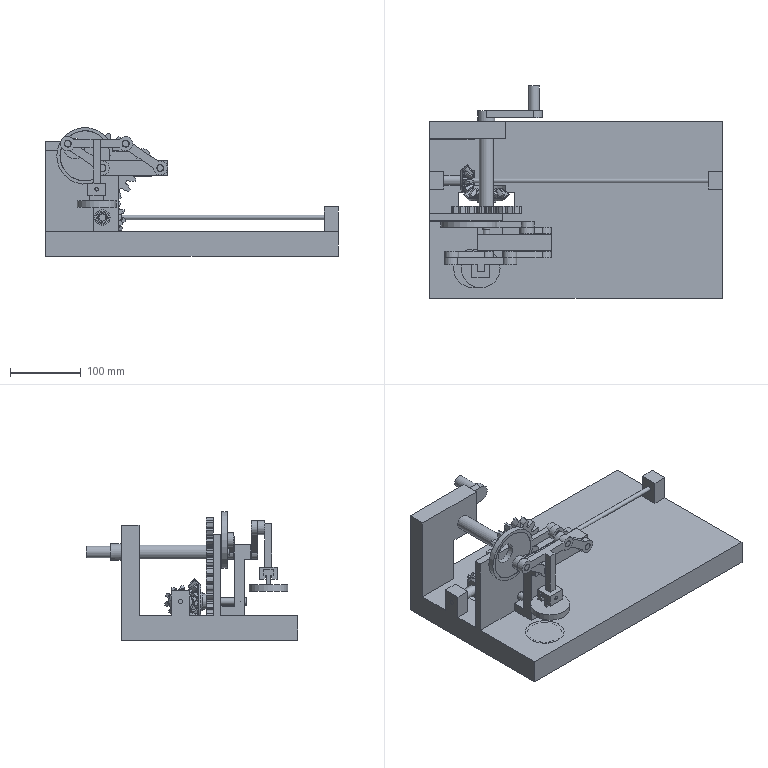Assembly | NX | mm | 25 component files | 69 solids | 907 faces | box 414.5 x 300 x 182.21 mm | volume 4371496 mm3 | spline 300 | plane 261 | cylinder 126 | other 90 | cone 84 | sphere 38 | torus 8 | commonest cylinder face diameters 10 x19 77.5 x18 20 x15 37.46 x10 16 x6 14 x5 22 x5 6 x4
Bill of materials:
unnamed part 1 | 1 |  | Short cylinder with a thin, slightly larger flange or lip at one end, like a cap or plug shape.
unnamed part 2 | 1 |  | Stepped round shaft: a long small-diameter section, a short step, a middle-diameter section, a raised collar, then a larger-diameter section.
unnamed part 3 | 2 |  | Flat, slender link bar with a rounded eye at each end, each with a through-hole.
unnamed part 4 | 1 |  | Circular disc base with a raised upright block in the middle. From the side the block looks T-shaped, and its wider upper head has a horizontal through-hole.
unnamed part 5 | 1 |  | Crank-like part: a long round shaft with a small reduced-diameter tip at one end and a collar at the other end, joined to a flat arm with rounded ends. A short cylindrical pin sticks out from the far end of the arm, parallel to the shaft.
GB-T119.1-2000,10x18 | 3 |  | Parallel Pin, GB-T 119.1-2000,10x18
GB-T292_C-1994,71904_C | 2 |  | Open (unshielded) ball-bearing-like ring set: concentric outer and inner rings with 12 spherical balls evenly spaced in the annular gap; large bore relative to outer diameter, thin ring cross-section, short axial width.
GB-T119.1-2000,10x40 | 1 |  | Parallel Pin, GB-T 119.1-2000,10x40
unnamed part 6 | 1 |  | Short, thick, flat link with two rounded eye ends, each with a fairly large through-hole.
unnamed part 7 | 1 |  | Stepped cylindrical pin with two diameters: a longer larger-diameter section and a shorter smaller-diameter section.
unnamed part 8 | 1 |  | Thin flat ring with one straight radial arm that ends in a small eyelet with a hole.
GB-T292_AC-1994,71900_AC | 2 |  | Open (unshielded) ball-bearing-like ring set: concentric outer and inner rings with 8 spherical balls evenly spaced in the annular gap; smaller bore relative to outer diameter and proportionally larger balls than unnamed part.
unnamed part 9 | 1 |  | Straight-toothed bevel gear with a central through-bore and a short cylindrical hub on the back face.
unnamed part 10 | 1 |  | T-shaped link. A crossbar with a holed round eye at each end sits on top of a straight stem, and the stem ends in a rectangular block with a small cross-hole and a C-shaped slot that is open on one side.
unnamed part 11 | 1 |  | Two flat spur gears in the same plane with their teeth meshing: a larger gear (about 18 teeth) and a smaller gear (about 11 teeth), each with a central bore.
unnamed part 12 | 1 |  | Long, thin, straight cylindrical rod with plain ends.
unnamed part 13 | 1 |  | Rectangular base plate with a large round through-hole near one corner, several upright tabs/brackets with small holes clustered at one end, and a small upright tab with a small hole near the opposite edge.
GB-T119.1-2000,5x24 | 1 |  | Parallel Pin, GB-T 119.1-2000,5x24
unnamed part 14 | 1 |  | Small conical toothed gear (bevel-gear-like) with a plain cylindrical shaft sticking out from its back face and a small central bore at the toothed end.
unnamed part 15 | 1 |  | Flat circular disc with two round through-holes of different sizes, both off-center: one large hole near the edge and one small hole near the opposite side of the rim.
Mates:
1. fix | base 1 component
2. concentric | connecting_rod_bracket 1 edge | connecting_rod 1 edge
3. concentric | connecting_rod_bracket 1 edge | connecting_rod 2 edge
4. touch align | connecting_rod 1 face | base 1 edge
5. concentric | connecting_rod 2 edge | base 1 edge
6. concentric | stamp_holder 1 edge | connecting_rod_bracket 1 edge
7. concentric | connecting_rod_2 1 edge | base 1 edge
8. concentric | eccentric 1 edge | eccentric_rod 1 edge
9. concentric | eccentric_rod 1 edge | connecting_rod_2 1 edge
10. touch align | eccentric 1 face | base 1 face
11. concentric | spur_gear_set 1 edge | base 1 edge
12. concentric | drive_shaft 1 edge | spur_gear_set 1 edge
13. touch align | bevel_gear_2 1 face | long_shaft 1 face
14. touch align | drive_shaft 1 face | bevel_gear_1 1 face
15. distance | bevel_gear_1 1 face | drive_shaft 1 face
16. distance | bevel_gear_2 1 face | base 1 face
17. parallel | connecting_rod_bracket 1 face | eccentric_rod 1 face
18. parallel | eccentric_rod 1 face | base 1 face
19. concentric | GB-T292_AC-1994_71900_AC 2 edge | base 1 edge
20. concentric | GB-T292_AC-1994_71900_AC 1 edge | base 1 edge
21. concentric | GB-T292_C-1994_71904_C 2 edge | base 1 edge
22. concentric | GB-T292_C-1994_71904_C 1 edge | base 1 edge
23. concentric | rocker 1 edge | eccentric 1 edge
24. parallel | connecting_rod_2 1 face | connecting_rod 2 face
25. concentric | GB-T119_1-2000_10x18 1 edge | connecting_rod_bracket 1 edge
26. concentric | GB-T119_1-2000_10x18 2 edge | eccentric_rod 1 edge
27. concentric | GB-T119_1-2000_10x18 3 edge | connecting_rod_bracket 1 edge
28. concentric | GB-T119_1-2000_10x40 1 edge | connecting_rod 2 edge